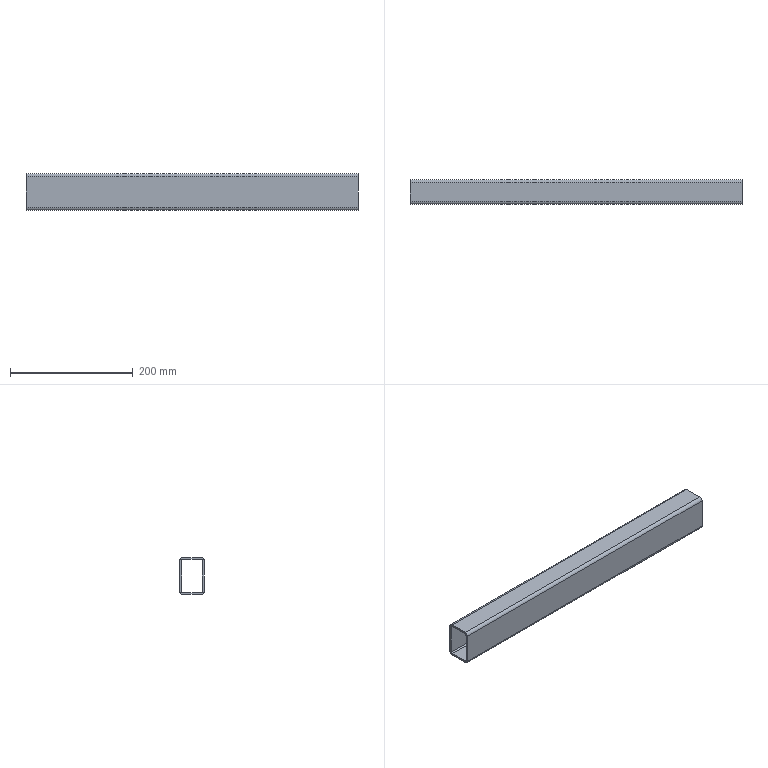Component | SolidWorks | THK-B1017FrontCrossBeam-2 | 1 solid | 22 faces | box 540 x 40 x 60 mm | volume 294774 mm3 | cylinder 12 | plane 10 | commonest cylinder face diameters 3.3 x4 10 x4 4 x4 | material Q235A
build123d program:
from build123d import *

# Parameters (mm, degrees)
EXTRUDE_THIN1_DEPTH   = 270
M4_TAPPED_HOLE1_D     = 3.3
M4_TAPPED_HOLE1_DEPTH = 3


with BuildPart() as part:
    # Sketch1 → Extrude-Thin1 (new, symmetric)
    with BuildSketch(Plane(origin=(0, 0, 0), x_dir=(0, 0, -1), z_dir=(1, 0, 0))):
        with BuildLine():
            Line((-30, 15), (-30, -15))
            ThreePointArc((-30, -15), (-28.536, -18.536), (-25, -20))
            Line((-25, -20), (25, -20))
            ThreePointArc((25, -20), (28.536, -18.536), (30, -15))
            Line((30, -15), (30, 15))
            ThreePointArc((30, 15), (28.536, 18.536), (25, 20))
            Line((25, 20), (-25, 20))
            ThreePointArc((-25, 20), (-28.536, 18.536), (-30, 15))
        make_face()
        with BuildLine():
            Line((-27, 15), (-27, -15))
            ThreePointArc((-27, -15), (-26.414, -16.414), (-25, -17))
            Line((-25, -17), (25, -17))
            ThreePointArc((25, -17), (26.414, -16.414), (27, -15))
            Line((27, -15), (27, 15))
            ThreePointArc((27, 15), (26.414, 16.414), (25, 17))
            Line((25, 17), (-25, 17))
            ThreePointArc((-25, 17), (-26.414, 16.414), (-27, 15))
        make_face(mode=Mode.SUBTRACT)
    extrude(amount=EXTRUDE_THIN1_DEPTH, both=True)

    # M4 Tapped Hole1
    with Locations(Plane(origin=(0, 20, 0), x_dir=(1, 0, 0), z_dir=(0, 1, 0))):
        with Locations((-150, 0), (-170, 0)):
            Hole(M4_TAPPED_HOLE1_D / 2, depth=M4_TAPPED_HOLE1_DEPTH)


solid = part.part

# Placed as in the assembly
solid = solid.moved(Location((0, -130, -860), (0, 0, 0)))
STEP:
#1=COLOUR_RGB('',0.7922,0.8196,0.9333);
#2=FILL_AREA_STYLE_COLOUR('',#1);
#3=FILL_AREA_STYLE('',(#2));
#4=SURFACE_STYLE_FILL_AREA(#3);
#5=SURFACE_SIDE_STYLE('',(#4));
#6=SURFACE_STYLE_USAGE(.BOTH.,#5);
#7=PRESENTATION_STYLE_ASSIGNMENT((#6));
#8=CARTESIAN_POINT('',(-5.906,-4.449,-33.793));
#9=VERTEX_POINT('',#8);
#10=CARTESIAN_POINT('',(-5.906,-4.449,-33.923));
#11=VERTEX_POINT('',#10);
#12=CARTESIAN_POINT('',(-5.906,-4.449,-33.858));
#13=DIRECTION('',(0.,-1.,0.));
#14=DIRECTION('',(0.,0.,-1.));
#15=AXIS2_PLACEMENT_3D('',#12,#13,#14);
#16=CIRCLE('',#15,0.06496);
#17=EDGE_CURVE('',#9,#11,#16,.T.);
#18=ORIENTED_EDGE('',*,*,#17,.T.);
#19=CARTESIAN_POINT('',(-5.906,-4.331,-33.923));
#20=VERTEX_POINT('',#19);
#21=CARTESIAN_POINT('',(-5.906,-4.331,-33.923));
#22=DIRECTION('',(0.,1.,0.));
#23=VECTOR('',#22,39.37);
#24=LINE('',#21,#23);
#25=EDGE_CURVE('',#11,#20,#24,.T.);
#26=ORIENTED_EDGE('',*,*,#25,.T.);
#27=CARTESIAN_POINT('',(-5.906,-4.331,-33.793));
#28=VERTEX_POINT('',#27);
#29=CARTESIAN_POINT('',(-5.906,-4.331,-33.858));
#30=DIRECTION('',(0.,1.,0.));
#31=DIRECTION('',(0.,0.,1.));
#32=AXIS2_PLACEMENT_3D('',#29,#30,#31);
#33=CIRCLE('',#32,0.06496);
#34=EDGE_CURVE('',#20,#28,#33,.T.);
#35=ORIENTED_EDGE('',*,*,#34,.T.);
#36=CARTESIAN_POINT('',(-5.906,-4.331,-33.793));
#37=DIRECTION('',(0.,1.,0.));
#38=VECTOR('',#37,39.37);
#39=LINE('',#36,#38);
#40=EDGE_CURVE('',#9,#28,#39,.T.);
#41=ORIENTED_EDGE('',*,*,#40,.F.);
#42=EDGE_LOOP('',(#18,#26,#35,#41));
#43=FACE_OUTER_BOUND('',#42,.T.);
#44=CARTESIAN_POINT('',(-5.906,-4.331,-33.858));
#45=DIRECTION('',(0.,1.,0.));
#46=DIRECTION('',(0.,0.,1.));
#47=AXIS2_PLACEMENT_3D('',#44,#45,#46);
#48=CYLINDRICAL_SURFACE('',#47,0.06496);
#49=ADVANCED_FACE('',(#43),#48,.F.);
#50=CARTESIAN_POINT('',(-6.693,-4.449,-33.793));
#51=VERTEX_POINT('',#50);
#52=CARTESIAN_POINT('',(-6.693,-4.449,-33.923));
#53=VERTEX_POINT('',#52);
#54=CARTESIAN_POINT('',(-6.693,-4.449,-33.858));
#55=DIRECTION('',(0.,-1.,0.));
#56=DIRECTION('',(0.,0.,-1.));
#57=AXIS2_PLACEMENT_3D('',#54,#55,#56);
#58=CIRCLE('',#57,0.06496);
#59=EDGE_CURVE('',#51,#53,#58,.T.);
#60=ORIENTED_EDGE('',*,*,#59,.T.);
#61=CARTESIAN_POINT('',(-6.693,-4.331,-33.923));
#62=VERTEX_POINT('',#61);
#63=CARTESIAN_POINT('',(-6.693,-4.331,-33.923));
#64=DIRECTION('',(0.,1.,0.));
#65=VECTOR('',#64,39.37);
#66=LINE('',#63,#65);
#67=EDGE_CURVE('',#53,#62,#66,.T.);
#68=ORIENTED_EDGE('',*,*,#67,.T.);
#69=CARTESIAN_POINT('',(-6.693,-4.331,-33.793));
#70=VERTEX_POINT('',#69);
#71=CARTESIAN_POINT('',(-6.693,-4.331,-33.858));
#72=DIRECTION('',(0.,1.,0.));
#73=DIRECTION('',(0.,0.,1.));
#74=AXIS2_PLACEMENT_3D('',#71,#72,#73);
#75=CIRCLE('',#74,0.06496);
#76=EDGE_CURVE('',#62,#70,#75,.T.);
#77=ORIENTED_EDGE('',*,*,#76,.T.);
#78=CARTESIAN_POINT('',(-6.693,-4.331,-33.793));
#79=DIRECTION('',(0.,1.,0.));
#80=VECTOR('',#79,39.37);
#81=LINE('',#78,#80);
#82=EDGE_CURVE('',#51,#70,#81,.T.);
#83=ORIENTED_EDGE('',*,*,#82,.F.);
#84=EDGE_LOOP('',(#60,#68,#77,#83));
#85=FACE_OUTER_BOUND('',#84,.T.);
#86=CARTESIAN_POINT('',(-6.693,-4.331,-33.858));
#87=DIRECTION('',(0.,1.,0.));
#88=DIRECTION('',(0.,0.,1.));
#89=AXIS2_PLACEMENT_3D('',#86,#87,#88);
#90=CYLINDRICAL_SURFACE('',#89,0.06496);
#91=ADVANCED_FACE('',(#85),#90,.F.);
#92=CARTESIAN_POINT('',(10.63,-5.709,-32.677));
#93=VERTEX_POINT('',#92);
#94=CARTESIAN_POINT('',(10.63,-5.906,-32.874));
#95=VERTEX_POINT('',#94);
#96=CARTESIAN_POINT('',(10.63,-5.709,-32.874));
#97=DIRECTION('',(1.,0.,0.));
#98=DIRECTION('',(0.,0.,-1.));
#99=AXIS2_PLACEMENT_3D('',#96,#97,#98);
#100=CIRCLE('',#99,0.1969);
#101=EDGE_CURVE('',#93,#95,#100,.T.);
#102=ORIENTED_EDGE('',*,*,#101,.T.);
#103=CARTESIAN_POINT('',(10.63,-5.906,-34.843));
#104=VERTEX_POINT('',#103);
#105=CARTESIAN_POINT('',(10.63,-5.906,-32.874));
#106=DIRECTION('',(0.,0.,-1.));
#107=VECTOR('',#106,39.37);
#108=LINE('',#105,#107);
#109=EDGE_CURVE('',#95,#104,#108,.T.);
#110=ORIENTED_EDGE('',*,*,#109,.T.);
#111=CARTESIAN_POINT('',(10.63,-5.709,-35.039));
#112=VERTEX_POINT('',#111);
#113=CARTESIAN_POINT('',(10.63,-5.709,-34.843));
#114=DIRECTION('',(1.,0.,0.));
#115=DIRECTION('',(0.,0.,1.));
#116=AXIS2_PLACEMENT_3D('',#113,#114,#115);
#117=CIRCLE('',#116,0.1969);
#118=EDGE_CURVE('',#104,#112,#117,.T.);
#119=ORIENTED_EDGE('',*,*,#118,.T.);
#120=CARTESIAN_POINT('',(10.63,-4.528,-35.039));
#121=VERTEX_POINT('',#120);
#122=CARTESIAN_POINT('',(10.63,-5.709,-35.039));
#123=DIRECTION('',(0.,1.,0.));
#124=VECTOR('',#123,39.37);
#125=LINE('',#122,#124);
#126=EDGE_CURVE('',#112,#121,#125,.T.);
#127=ORIENTED_EDGE('',*,*,#126,.T.);
#128=CARTESIAN_POINT('',(10.63,-4.331,-34.843));
#129=VERTEX_POINT('',#128);
#130=CARTESIAN_POINT('',(10.63,-4.528,-34.843));
#131=DIRECTION('',(1.,0.,0.));
#132=DIRECTION('',(0.,0.,-1.));
#133=AXIS2_PLACEMENT_3D('',#130,#131,#132);
#134=CIRCLE('',#133,0.1969);
#135=EDGE_CURVE('',#121,#129,#134,.T.);
#136=ORIENTED_EDGE('',*,*,#135,.T.);
#137=CARTESIAN_POINT('',(10.63,-4.331,-32.874));
#138=VERTEX_POINT('',#137);
#139=CARTESIAN_POINT('',(10.63,-4.331,-32.874));
#140=DIRECTION('',(0.,0.,1.));
#141=VECTOR('',#140,39.37);
#142=LINE('',#139,#141);
#143=EDGE_CURVE('',#129,#138,#142,.T.);
#144=ORIENTED_EDGE('',*,*,#143,.T.);
#145=CARTESIAN_POINT('',(10.63,-4.528,-32.677));
#146=VERTEX_POINT('',#145);
#147=CARTESIAN_POINT('',(10.63,-4.528,-32.874));
#148=DIRECTION('',(1.,0.,0.));
#149=DIRECTION('',(0.,0.,1.));
#150=AXIS2_PLACEMENT_3D('',#147,#148,#149);
#151=CIRCLE('',#150,0.1969);
#152=EDGE_CURVE('',#138,#146,#151,.T.);
#153=ORIENTED_EDGE('',*,*,#152,.T.);
#154=CARTESIAN_POINT('',(10.63,-5.709,-32.677));
#155=DIRECTION('',(0.,-1.,0.));
#156=VECTOR('',#155,39.37);
#157=LINE('',#154,#156);
#158=EDGE_CURVE('',#146,#93,#157,.T.);
#159=ORIENTED_EDGE('',*,*,#158,.T.);
#160=EDGE_LOOP('',(#102,#110,#119,#127,#136,#144,#153,#159));
#161=FACE_OUTER_BOUND('',#160,.T.);
#162=CARTESIAN_POINT('',(10.63,-5.787,-32.874));
#163=VERTEX_POINT('',#162);
#164=CARTESIAN_POINT('',(10.63,-5.787,-34.843));
#165=VERTEX_POINT('',#164);
#166=CARTESIAN_POINT('',(10.63,-5.787,-32.874));
#167=DIRECTION('',(0.,0.,-1.));
#168=VECTOR('',#167,39.37);
#169=LINE('',#166,#168);
#170=EDGE_CURVE('',#163,#165,#169,.T.);
#171=ORIENTED_EDGE('',*,*,#170,.F.);
#172=CARTESIAN_POINT('',(10.63,-5.709,-32.795));
#173=VERTEX_POINT('',#172);
#174=CARTESIAN_POINT('',(10.63,-5.709,-32.874));
#175=DIRECTION('',(1.,0.,0.));
#176=DIRECTION('',(0.,0.,-1.));
#177=AXIS2_PLACEMENT_3D('',#174,#175,#176);
#178=CIRCLE('',#177,0.07874);
#179=EDGE_CURVE('',#173,#163,#178,.T.);
#180=ORIENTED_EDGE('',*,*,#179,.F.);
#181=CARTESIAN_POINT('',(10.63,-4.528,-32.795));
#182=VERTEX_POINT('',#181);
#183=CARTESIAN_POINT('',(10.63,-5.709,-32.795));
#184=DIRECTION('',(0.,-1.,0.));
#185=VECTOR('',#184,39.37);
#186=LINE('',#183,#185);
#187=EDGE_CURVE('',#182,#173,#186,.T.);
#188=ORIENTED_EDGE('',*,*,#187,.F.);
#189=CARTESIAN_POINT('',(10.63,-4.449,-32.874));
#190=VERTEX_POINT('',#189);
#191=CARTESIAN_POINT('',(10.63,-4.528,-32.874));
#192=DIRECTION('',(1.,0.,0.));
#193=DIRECTION('',(0.,0.,-1.));
#194=AXIS2_PLACEMENT_3D('',#191,#192,#193);
#195=CIRCLE('',#194,0.07874);
#196=EDGE_CURVE('',#190,#182,#195,.T.);
#197=ORIENTED_EDGE('',*,*,#196,.F.);
#198=CARTESIAN_POINT('',(10.63,-4.449,-34.843));
#199=VERTEX_POINT('',#198);
#200=CARTESIAN_POINT('',(10.63,-4.449,-32.874));
#201=DIRECTION('',(0.,0.,1.));
#202=VECTOR('',#201,39.37);
#203=LINE('',#200,#202);
#204=EDGE_CURVE('',#199,#190,#203,.T.);
#205=ORIENTED_EDGE('',*,*,#204,.F.);
#206=CARTESIAN_POINT('',(10.63,-4.528,-34.921));
#207=VERTEX_POINT('',#206);
#208=CARTESIAN_POINT('',(10.63,-4.528,-34.843));
#209=DIRECTION('',(1.,0.,0.));
#210=DIRECTION('',(0.,0.,-1.));
#211=AXIS2_PLACEMENT_3D('',#208,#209,#210);
#212=CIRCLE('',#211,0.07874);
#213=EDGE_CURVE('',#207,#199,#212,.T.);
#214=ORIENTED_EDGE('',*,*,#213,.F.);
#215=CARTESIAN_POINT('',(10.63,-5.709,-34.921));
#216=VERTEX_POINT('',#215);
#217=CARTESIAN_POINT('',(10.63,-5.709,-34.921));
#218=DIRECTION('',(0.,1.,0.));
#219=VECTOR('',#218,39.37);
#220=LINE('',#217,#219);
#221=EDGE_CURVE('',#216,#207,#220,.T.);
#222=ORIENTED_EDGE('',*,*,#221,.F.);
#223=CARTESIAN_POINT('',(10.63,-5.709,-34.843));
#224=DIRECTION('',(1.,0.,0.));
#225=DIRECTION('',(0.,0.,-1.));
#226=AXIS2_PLACEMENT_3D('',#223,#224,#225);
#227=CIRCLE('',#226,0.07874);
#228=EDGE_CURVE('',#165,#216,#227,.T.);
#229=ORIENTED_EDGE('',*,*,#228,.F.);
#230=EDGE_LOOP('',(#171,#180,#188,#197,#205,#214,#222,#229));
#231=FACE_BOUND('',#230,.T.);
#232=CARTESIAN_POINT('',(10.63,-5.709,-32.874));
#233=DIRECTION('',(1.,0.,0.));
#234=DIRECTION('',(0.,0.,-1.));
#235=AXIS2_PLACEMENT_3D('',#232,#233,#234);
#236=PLANE('',#235);
#237=ADVANCED_FACE('',(#161,#231),#236,.T.);
#238=CARTESIAN_POINT('',(-10.63,-5.709,-32.677));
#239=VERTEX_POINT('',#238);
#240=CARTESIAN_POINT('',(-10.63,-5.906,-32.874));
#241=VERTEX_POINT('',#240);
#242=CARTESIAN_POINT('',(-10.63,-5.709,-32.874));
#243=DIRECTION('',(1.,0.,0.));
#244=DIRECTION('',(0.,0.,-1.));
#245=AXIS2_PLACEMENT_3D('',#242,#243,#244);
#246=CIRCLE('',#245,0.1969);
#247=EDGE_CURVE('',#239,#241,#246,.T.);
#248=ORIENTED_EDGE('',*,*,#247,.F.);
#249=CARTESIAN_POINT('',(-10.63,-4.528,-32.677));
#250=VERTEX_POINT('',#249);
#251=CARTESIAN_POINT('',(-10.63,-5.709,-32.677));
#252=DIRECTION('',(0.,-1.,0.));
#253=VECTOR('',#252,39.37);
#254=LINE('',#251,#253);
#255=EDGE_CURVE('',#250,#239,#254,.T.);
#256=ORIENTED_EDGE('',*,*,#255,.F.);
#257=CARTESIAN_POINT('',(-10.63,-4.331,-32.874));
#258=VERTEX_POINT('',#257);
#259=CARTESIAN_POINT('',(-10.63,-4.528,-32.874));
#260=DIRECTION('',(1.,0.,0.));
#261=DIRECTION('',(0.,0.,1.));
#262=AXIS2_PLACEMENT_3D('',#259,#260,#261);
#263=CIRCLE('',#262,0.1969);
#264=EDGE_CURVE('',#258,#250,#263,.T.);
#265=ORIENTED_EDGE('',*,*,#264,.F.);
#266=CARTESIAN_POINT('',(-10.63,-4.331,-34.843));
#267=VERTEX_POINT('',#266);
#268=CARTESIAN_POINT('',(-10.63,-4.331,-32.874));
#269=DIRECTION('',(0.,0.,1.));
#270=VECTOR('',#269,39.37);
#271=LINE('',#268,#270);
#272=EDGE_CURVE('',#267,#258,#271,.T.);
#273=ORIENTED_EDGE('',*,*,#272,.F.);
#274=CARTESIAN_POINT('',(-10.63,-4.528,-35.039));
#275=VERTEX_POINT('',#274);
#276=CARTESIAN_POINT('',(-10.63,-4.528,-34.843));
#277=DIRECTION('',(1.,0.,0.));
#278=DIRECTION('',(0.,0.,-1.));
#279=AXIS2_PLACEMENT_3D('',#276,#277,#278);
#280=CIRCLE('',#279,0.1969);
#281=EDGE_CURVE('',#275,#267,#280,.T.);
#282=ORIENTED_EDGE('',*,*,#281,.F.);
#283=CARTESIAN_POINT('',(-10.63,-5.709,-35.039));
#284=VERTEX_POINT('',#283);
#285=CARTESIAN_POINT('',(-10.63,-5.709,-35.039));
#286=DIRECTION('',(0.,1.,0.));
#287=VECTOR('',#286,39.37);
#288=LINE('',#285,#287);
#289=EDGE_CURVE('',#284,#275,#288,.T.);
#290=ORIENTED_EDGE('',*,*,#289,.F.);
#291=CARTESIAN_POINT('',(-10.63,-5.906,-34.843));
#292=VERTEX_POINT('',#291);
#293=CARTESIAN_POINT('',(-10.63,-5.709,-34.843));
#294=DIRECTION('',(1.,0.,0.));
#295=DIRECTION('',(0.,0.,1.));
#296=AXIS2_PLACEMENT_3D('',#293,#294,#295);
#297=CIRCLE('',#296,0.1969);
#298=EDGE_CURVE('',#292,#284,#297,.T.);
#299=ORIENTED_EDGE('',*,*,#298,.F.);
#300=CARTESIAN_POINT('',(-10.63,-5.906,-32.874));
#301=DIRECTION('',(0.,0.,-1.));
#302=VECTOR('',#301,39.37);
#303=LINE('',#300,#302);
#304=EDGE_CURVE('',#241,#292,#303,.T.);
#305=ORIENTED_EDGE('',*,*,#304,.F.);
#306=EDGE_LOOP('',(#248,#256,#265,#273,#282,#290,#299,#305));
#307=FACE_OUTER_BOUND('',#306,.T.);
#308=CARTESIAN_POINT('',(-10.63,-5.709,-32.795));
#309=VERTEX_POINT('',#308);
#310=CARTESIAN_POINT('',(-10.63,-5.787,-32.874));
#311=VERTEX_POINT('',#310);
#312=CARTESIAN_POINT('',(-10.63,-5.709,-32.874));
#313=DIRECTION('',(1.,0.,0.));
#314=DIRECTION('',(0.,0.,-1.));
#315=AXIS2_PLACEMENT_3D('',#312,#313,#314);
#316=CIRCLE('',#315,0.07874);
#317=EDGE_CURVE('',#309,#311,#316,.T.);
#318=ORIENTED_EDGE('',*,*,#317,.T.);
#319=CARTESIAN_POINT('',(-10.63,-5.787,-34.843));
#320=VERTEX_POINT('',#319);
#321=CARTESIAN_POINT('',(-10.63,-5.787,-32.874));
#322=DIRECTION('',(0.,0.,-1.));
#323=VECTOR('',#322,39.37);
#324=LINE('',#321,#323);
#325=EDGE_CURVE('',#311,#320,#324,.T.);
#326=ORIENTED_EDGE('',*,*,#325,.T.);
#327=CARTESIAN_POINT('',(-10.63,-5.709,-34.921));
#328=VERTEX_POINT('',#327);
#329=CARTESIAN_POINT('',(-10.63,-5.709,-34.843));
#330=DIRECTION('',(1.,0.,0.));
#331=DIRECTION('',(0.,0.,-1.));
#332=AXIS2_PLACEMENT_3D('',#329,#330,#331);
#333=CIRCLE('',#332,0.07874);
#334=EDGE_CURVE('',#320,#328,#333,.T.);
#335=ORIENTED_EDGE('',*,*,#334,.T.);
#336=CARTESIAN_POINT('',(-10.63,-4.528,-34.921));
#337=VERTEX_POINT('',#336);
#338=CARTESIAN_POINT('',(-10.63,-5.709,-34.921));
#339=DIRECTION('',(0.,1.,0.));
#340=VECTOR('',#339,39.37);
#341=LINE('',#338,#340);
#342=EDGE_CURVE('',#328,#337,#341,.T.);
#343=ORIENTED_EDGE('',*,*,#342,.T.);
#344=CARTESIAN_POINT('',(-10.63,-4.449,-34.843));
#345=VERTEX_POINT('',#344);
#346=CARTESIAN_POINT('',(-10.63,-4.528,-34.843));
#347=DIRECTION('',(1.,0.,0.));
#348=DIRECTION('',(0.,0.,-1.));
#349=AXIS2_PLACEMENT_3D('',#346,#347,#348);
#350=CIRCLE('',#349,0.07874);
#351=EDGE_CURVE('',#337,#345,#350,.T.);
#352=ORIENTED_EDGE('',*,*,#351,.T.);
#353=CARTESIAN_POINT('',(-10.63,-4.449,-32.874));
#354=VERTEX_POINT('',#353);
#355=CARTESIAN_POINT('',(-10.63,-4.449,-32.874));
#356=DIRECTION('',(0.,0.,1.));
#357=VECTOR('',#356,39.37);
#358=LINE('',#355,#357);
#359=EDGE_CURVE('',#345,#354,#358,.T.);
#360=ORIENTED_EDGE('',*,*,#359,.T.);
#361=CARTESIAN_POINT('',(-10.63,-4.528,-32.795));
#362=VERTEX_POINT('',#361);
#363=CARTESIAN_POINT('',(-10.63,-4.528,-32.874));
#364=DIRECTION('',(1.,0.,0.));
#365=DIRECTION('',(0.,0.,-1.));
#366=AXIS2_PLACEMENT_3D('',#363,#364,#365);
#367=CIRCLE('',#366,0.07874);
#368=EDGE_CURVE('',#354,#362,#367,.T.);
#369=ORIENTED_EDGE('',*,*,#368,.T.);
#370=CARTESIAN_POINT('',(-10.63,-5.709,-32.795));
#371=DIRECTION('',(0.,-1.,0.));
#372=VECTOR('',#371,39.37);
#373=LINE('',#370,#372);
#374=EDGE_CURVE('',#362,#309,#373,.T.);
#375=ORIENTED_EDGE('',*,*,#374,.T.);
#376=EDGE_LOOP('',(#318,#326,#335,#343,#352,#360,#369,#375));
#377=FACE_BOUND('',#376,.T.);
#378=CARTESIAN_POINT('',(-10.63,-5.709,-32.874));
#379=DIRECTION('',(1.,0.,0.));
#380=DIRECTION('',(0.,0.,-1.));
#381=AXIS2_PLACEMENT_3D('',#378,#379,#380);
#382=PLANE('',#381);
#383=ADVANCED_FACE('',(#307,#377),#382,.F.);
#384=ORIENTED_EDGE('',*,*,#247,.T.);
#385=CARTESIAN_POINT('',(10.63,-5.906,-32.874));
#386=DIRECTION('',(-1.,0.,0.));
#387=VECTOR('',#386,39.37);
#388=LINE('',#385,#387);
#389=EDGE_CURVE('',#95,#241,#388,.T.);
#390=ORIENTED_EDGE('',*,*,#389,.F.);
#391=ORIENTED_EDGE('',*,*,#101,.F.);
#392=CARTESIAN_POINT('',(10.63,-5.709,-32.677));
#393=DIRECTION('',(-1.,0.,0.));
#394=VECTOR('',#393,39.37);
#395=LINE('',#392,#394);
#396=EDGE_CURVE('',#93,#239,#395,.T.);
#397=ORIENTED_EDGE('',*,*,#396,.T.);
#398=EDGE_LOOP('',(#384,#390,#391,#397));
#399=FACE_OUTER_BOUND('',#398,.T.);
#400=CARTESIAN_POINT('',(10.63,-5.709,-32.874));
#401=DIRECTION('',(-1.,0.,0.));
#402=DIRECTION('',(0.,0.,1.));
#403=AXIS2_PLACEMENT_3D('',#400,#401,#402);
#404=CYLINDRICAL_SURFACE('',#403,0.1969);
#405=ADVANCED_FACE('',(#399),#404,.T.);
#406=ORIENTED_EDGE('',*,*,#304,.T.);
#407=CARTESIAN_POINT('',(10.63,-5.906,-34.843));
#408=DIRECTION('',(-1.,0.,0.));
#409=VECTOR('',#408,39.37);
#410=LINE('',#407,#409);
#411=EDGE_CURVE('',#104,#292,#410,.T.);
#412=ORIENTED_EDGE('',*,*,#411,.F.);
#413=ORIENTED_EDGE('',*,*,#109,.F.);
#414=ORIENTED_EDGE('',*,*,#389,.T.);
#415=EDGE_LOOP('',(#406,#412,#413,#414));
#416=FACE_OUTER_BOUND('',#415,.T.);
#417=CARTESIAN_POINT('',(10.63,-5.906,-32.874));
#418=DIRECTION('',(0.,1.,0.));
#419=DIRECTION('',(0.,0.,1.));
#420=AXIS2_PLACEMENT_3D('',#417,#418,#419);
#421=PLANE('',#420);
#422=ADVANCED_FACE('',(#416),#421,.F.);
#423=ORIENTED_EDGE('',*,*,#298,.T.);
#424=CARTESIAN_POINT('',(10.63,-5.709,-35.039));
#425=DIRECTION('',(-1.,0.,0.));
#426=VECTOR('',#425,39.37);
#427=LINE('',#424,#426);
#428=EDGE_CURVE('',#112,#284,#427,.T.);
#429=ORIENTED_EDGE('',*,*,#428,.F.);
#430=ORIENTED_EDGE('',*,*,#118,.F.);
#431=ORIENTED_EDGE('',*,*,#411,.T.);
#432=EDGE_LOOP('',(#423,#429,#430,#431));
#433=FACE_OUTER_BOUND('',#432,.T.);
#434=CARTESIAN_POINT('',(10.63,-5.709,-34.843));
#435=DIRECTION('',(-1.,0.,0.));
#436=DIRECTION('',(0.,0.,1.));
#437=AXIS2_PLACEMENT_3D('',#434,#435,#436);
#438=CYLINDRICAL_SURFACE('',#437,0.1969);
#439=ADVANCED_FACE('',(#433),#438,.T.);
#440=ORIENTED_EDGE('',*,*,#289,.T.);
#441=CARTESIAN_POINT('',(10.63,-4.528,-35.039));
#442=DIRECTION('',(-1.,0.,0.));
#443=VECTOR('',#442,39.37);
#444=LINE('',#441,#443);
#445=EDGE_CURVE('',#121,#275,#444,.T.);
#446=ORIENTED_EDGE('',*,*,#445,.F.);
#447=ORIENTED_EDGE('',*,*,#126,.F.);
#448=ORIENTED_EDGE('',*,*,#428,.T.);
#449=EDGE_LOOP('',(#440,#446,#447,#448));
#450=FACE_OUTER_BOUND('',#449,.T.);
#451=CARTESIAN_POINT('',(10.63,-5.709,-35.039));
#452=DIRECTION('',(0.,0.,1.));
#453=DIRECTION('',(1.,0.,0.));
#454=AXIS2_PLACEMENT_3D('',#451,#452,#453);
#455=PLANE('',#454);
#456=ADVANCED_FACE('',(#450),#455,.F.);
#457=ORIENTED_EDGE('',*,*,#281,.T.);
#458=CARTESIAN_POINT('',(10.63,-4.331,-34.843));
#459=DIRECTION('',(-1.,0.,0.));
#460=VECTOR('',#459,39.37);
#461=LINE('',#458,#460);
#462=EDGE_CURVE('',#129,#267,#461,.T.);
#463=ORIENTED_EDGE('',*,*,#462,.F.);
#464=ORIENTED_EDGE('',*,*,#135,.F.);
#465=ORIENTED_EDGE('',*,*,#445,.T.);
#466=EDGE_LOOP('',(#457,#463,#464,#465));
#467=FACE_OUTER_BOUND('',#466,.T.);
#468=CARTESIAN_POINT('',(10.63,-4.528,-34.843));
#469=DIRECTION('',(-1.,0.,0.));
#470=DIRECTION('',(0.,0.,1.));
#471=AXIS2_PLACEMENT_3D('',#468,#469,#470);
#472=CYLINDRICAL_SURFACE('',#471,0.1969);
#473=ADVANCED_FACE('',(#467),#472,.T.);
#474=CARTESIAN_POINT('',(-5.906,-4.331,-33.858));
#475=DIRECTION('',(0.,1.,0.));
#476=DIRECTION('',(0.,0.,1.));
#477=AXIS2_PLACEMENT_3D('',#474,#475,#476);
#478=CIRCLE('',#477,0.06496);
#479=EDGE_CURVE('',#28,#20,#478,.T.);
#480=ORIENTED_EDGE('',*,*,#479,.F.);
#481=ORIENTED_EDGE('',*,*,#34,.F.);
#482=EDGE_LOOP('',(#480,#481));
#483=FACE_BOUND('',#482,.T.);
#484=CARTESIAN_POINT('',(-6.693,-4.331,-33.858));
#485=DIRECTION('',(0.,1.,0.));
#486=DIRECTION('',(0.,0.,1.));
#487=AXIS2_PLACEMENT_3D('',#484,#485,#486);
#488=CIRCLE('',#487,0.06496);
#489=EDGE_CURVE('',#70,#62,#488,.T.);
#490=ORIENTED_EDGE('',*,*,#489,.F.);
#491=ORIENTED_EDGE('',*,*,#76,.F.);
#492=EDGE_LOOP('',(#490,#491));
#493=FACE_BOUND('',#492,.T.);
#494=ORIENTED_EDGE('',*,*,#272,.T.);
#495=CARTESIAN_POINT('',(10.63,-4.331,-32.874));
#496=DIRECTION('',(-1.,0.,0.));
#497=VECTOR('',#496,39.37);
#498=LINE('',#495,#497);
#499=EDGE_CURVE('',#138,#258,#498,.T.);
#500=ORIENTED_EDGE('',*,*,#499,.F.);
#501=ORIENTED_EDGE('',*,*,#143,.F.);
#502=ORIENTED_EDGE('',*,*,#462,.T.);
#503=EDGE_LOOP('',(#494,#500,#501,#502));
#504=FACE_OUTER_BOUND('',#503,.T.);
#505=CARTESIAN_POINT('',(10.63,-4.331,-32.874));
#506=DIRECTION('',(0.,-1.,0.));
#507=DIRECTION('',(0.,0.,-1.));
#508=AXIS2_PLACEMENT_3D('',#505,#506,#507);
#509=PLANE('',#508);
#510=ADVANCED_FACE('',(#483,#493,#504),#509,.F.);
#511=ORIENTED_EDGE('',*,*,#264,.T.);
#512=CARTESIAN_POINT('',(10.63,-4.528,-32.677));
#513=DIRECTION('',(-1.,0.,0.));
#514=VECTOR('',#513,39.37);
#515=LINE('',#512,#514);
#516=EDGE_CURVE('',#146,#250,#515,.T.);
#517=ORIENTED_EDGE('',*,*,#516,.F.);
#518=ORIENTED_EDGE('',*,*,#152,.F.);
#519=ORIENTED_EDGE('',*,*,#499,.T.);
#520=EDGE_LOOP('',(#511,#517,#518,#519));
#521=FACE_OUTER_BOUND('',#520,.T.);
#522=CARTESIAN_POINT('',(10.63,-4.528,-32.874));
#523=DIRECTION('',(-1.,0.,0.));
#524=DIRECTION('',(0.,0.,1.));
#525=AXIS2_PLACEMENT_3D('',#522,#523,#524);
#526=CYLINDRICAL_SURFACE('',#525,0.1969);
#527=ADVANCED_FACE('',(#521),#526,.T.);
#528=ORIENTED_EDGE('',*,*,#255,.T.);
#529=ORIENTED_EDGE('',*,*,#396,.F.);
#530=ORIENTED_EDGE('',*,*,#158,.F.);
#531=ORIENTED_EDGE('',*,*,#516,.T.);
#532=EDGE_LOOP('',(#528,#529,#530,#531));
#533=FACE_OUTER_BOUND('',#532,.T.);
#534=CARTESIAN_POINT('',(10.63,-5.709,-32.677));
#535=DIRECTION('',(0.,0.,-1.));
#536=DIRECTION('',(-1.,0.,0.));
#537=AXIS2_PLACEMENT_3D('',#534,#535,#536);
#538=PLANE('',#537);
#539=ADVANCED_FACE('',(#533),#538,.F.);
#540=ORIENTED_EDGE('',*,*,#317,.F.);
#541=CARTESIAN_POINT('',(10.63,-5.709,-32.795));
#542=DIRECTION('',(-1.,0.,0.));
#543=VECTOR('',#542,39.37);
#544=LINE('',#541,#543);
#545=EDGE_CURVE('',#173,#309,#544,.T.);
#546=ORIENTED_EDGE('',*,*,#545,.F.);
#547=ORIENTED_EDGE('',*,*,#179,.T.);
#548=CARTESIAN_POINT('',(10.63,-5.787,-32.874));
#549=DIRECTION('',(-1.,0.,0.));
#550=VECTOR('',#549,39.37);
#551=LINE('',#548,#550);
#552=EDGE_CURVE('',#163,#311,#551,.T.);
#553=ORIENTED_EDGE('',*,*,#552,.T.);
#554=EDGE_LOOP('',(#540,#546,#547,#553));
#555=FACE_OUTER_BOUND('',#554,.T.);
#556=CARTESIAN_POINT('',(10.63,-5.709,-32.874));
#557=DIRECTION('',(-1.,0.,0.));
#558=DIRECTION('',(0.,0.,1.));
#559=AXIS2_PLACEMENT_3D('',#556,#557,#558);
#560=CYLINDRICAL_SURFACE('',#559,0.07874);
#561=ADVANCED_FACE('',(#555),#560,.F.);
#562=ORIENTED_EDGE('',*,*,#325,.F.);
#563=ORIENTED_EDGE('',*,*,#552,.F.);
#564=ORIENTED_EDGE('',*,*,#170,.T.);
#565=CARTESIAN_POINT('',(10.63,-5.787,-34.843));
#566=DIRECTION('',(-1.,0.,0.));
#567=VECTOR('',#566,39.37);
#568=LINE('',#565,#567);
#569=EDGE_CURVE('',#165,#320,#568,.T.);
#570=ORIENTED_EDGE('',*,*,#569,.T.);
#571=EDGE_LOOP('',(#562,#563,#564,#570));
#572=FACE_OUTER_BOUND('',#571,.T.);
#573=CARTESIAN_POINT('',(10.63,-5.787,-32.874));
#574=DIRECTION('',(0.,1.,0.));
#575=DIRECTION('',(0.,0.,1.));
#576=AXIS2_PLACEMENT_3D('',#573,#574,#575);
#577=PLANE('',#576);
#578=ADVANCED_FACE('',(#572),#577,.T.);
#579=ORIENTED_EDGE('',*,*,#334,.F.);
#580=ORIENTED_EDGE('',*,*,#569,.F.);
#581=ORIENTED_EDGE('',*,*,#228,.T.);
#582=CARTESIAN_POINT('',(10.63,-5.709,-34.921));
#583=DIRECTION('',(-1.,0.,0.));
#584=VECTOR('',#583,39.37);
#585=LINE('',#582,#584);
#586=EDGE_CURVE('',#216,#328,#585,.T.);
#587=ORIENTED_EDGE('',*,*,#586,.T.);
#588=EDGE_LOOP('',(#579,#580,#581,#587));
#589=FACE_OUTER_BOUND('',#588,.T.);
#590=CARTESIAN_POINT('',(10.63,-5.709,-34.843));
#591=DIRECTION('',(-1.,0.,0.));
#592=DIRECTION('',(0.,0.,1.));
#593=AXIS2_PLACEMENT_3D('',#590,#591,#592);
#594=CYLINDRICAL_SURFACE('',#593,0.07874);
#595=ADVANCED_FACE('',(#589),#594,.F.);
#596=ORIENTED_EDGE('',*,*,#342,.F.);
#597=ORIENTED_EDGE('',*,*,#586,.F.);
#598=ORIENTED_EDGE('',*,*,#221,.T.);
#599=CARTESIAN_POINT('',(10.63,-4.528,-34.921));
#600=DIRECTION('',(-1.,0.,0.));
#601=VECTOR('',#600,39.37);
#602=LINE('',#599,#601);
#603=EDGE_CURVE('',#207,#337,#602,.T.);
#604=ORIENTED_EDGE('',*,*,#603,.T.);
#605=EDGE_LOOP('',(#596,#597,#598,#604));
#606=FACE_OUTER_BOUND('',#605,.T.);
#607=CARTESIAN_POINT('',(10.63,-5.709,-34.921));
#608=DIRECTION('',(0.,0.,1.));
#609=DIRECTION('',(1.,0.,0.));
#610=AXIS2_PLACEMENT_3D('',#607,#608,#609);
#611=PLANE('',#610);
#612=ADVANCED_FACE('',(#606),#611,.T.);
#613=ORIENTED_EDGE('',*,*,#351,.F.);
#614=ORIENTED_EDGE('',*,*,#603,.F.);
#615=ORIENTED_EDGE('',*,*,#213,.T.);
#616=CARTESIAN_POINT('',(10.63,-4.449,-34.843));
#617=DIRECTION('',(-1.,0.,0.));
#618=VECTOR('',#617,39.37);
#619=LINE('',#616,#618);
#620=EDGE_CURVE('',#199,#345,#619,.T.);
#621=ORIENTED_EDGE('',*,*,#620,.T.);
#622=EDGE_LOOP('',(#613,#614,#615,#621));
#623=FACE_OUTER_BOUND('',#622,.T.);
#624=CARTESIAN_POINT('',(10.63,-4.528,-34.843));
#625=DIRECTION('',(-1.,0.,0.));
#626=DIRECTION('',(0.,0.,1.));
#627=AXIS2_PLACEMENT_3D('',#624,#625,#626);
#628=CYLINDRICAL_SURFACE('',#627,0.07874);
#629=ADVANCED_FACE('',(#623),#628,.F.);
#630=ORIENTED_EDGE('',*,*,#17,.F.);
#631=CARTESIAN_POINT('',(-5.906,-4.449,-33.858));
#632=DIRECTION('',(0.,-1.,0.));
#633=DIRECTION('',(0.,0.,-1.));
#634=AXIS2_PLACEMENT_3D('',#631,#632,#633);
#635=CIRCLE('',#634,0.06496);
#636=EDGE_CURVE('',#11,#9,#635,.T.);
#637=ORIENTED_EDGE('',*,*,#636,.F.);
#638=EDGE_LOOP('',(#630,#637));
#639=FACE_BOUND('',#638,.T.);
#640=ORIENTED_EDGE('',*,*,#59,.F.);
#641=CARTESIAN_POINT('',(-6.693,-4.449,-33.858));
#642=DIRECTION('',(0.,-1.,0.));
#643=DIRECTION('',(0.,0.,-1.));
#644=AXIS2_PLACEMENT_3D('',#641,#642,#643);
#645=CIRCLE('',#644,0.06496);
#646=EDGE_CURVE('',#53,#51,#645,.T.);
#647=ORIENTED_EDGE('',*,*,#646,.F.);
#648=EDGE_LOOP('',(#640,#647));
#649=FACE_BOUND('',#648,.T.);
#650=ORIENTED_EDGE('',*,*,#359,.F.);
#651=ORIENTED_EDGE('',*,*,#620,.F.);
#652=ORIENTED_EDGE('',*,*,#204,.T.);
#653=CARTESIAN_POINT('',(10.63,-4.449,-32.874));
#654=DIRECTION('',(-1.,0.,0.));
#655=VECTOR('',#654,39.37);
#656=LINE('',#653,#655);
#657=EDGE_CURVE('',#190,#354,#656,.T.);
#658=ORIENTED_EDGE('',*,*,#657,.T.);
#659=EDGE_LOOP('',(#650,#651,#652,#658));
#660=FACE_OUTER_BOUND('',#659,.T.);
#661=CARTESIAN_POINT('',(10.63,-4.449,-32.874));
#662=DIRECTION('',(0.,-1.,0.));
#663=DIRECTION('',(0.,0.,-1.));
#664=AXIS2_PLACEMENT_3D('',#661,#662,#663);
#665=PLANE('',#664);
#666=ADVANCED_FACE('',(#639,#649,#660),#665,.T.);
#667=ORIENTED_EDGE('',*,*,#368,.F.);
#668=ORIENTED_EDGE('',*,*,#657,.F.);
#669=ORIENTED_EDGE('',*,*,#196,.T.);
#670=CARTESIAN_POINT('',(10.63,-4.528,-32.795));
#671=DIRECTION('',(-1.,0.,0.));
#672=VECTOR('',#671,39.37);
#673=LINE('',#670,#672);
#674=EDGE_CURVE('',#182,#362,#673,.T.);
#675=ORIENTED_EDGE('',*,*,#674,.T.);
#676=EDGE_LOOP('',(#667,#668,#669,#675));
#677=FACE_OUTER_BOUND('',#676,.T.);
#678=CARTESIAN_POINT('',(10.63,-4.528,-32.874));
#679=DIRECTION('',(-1.,0.,0.));
#680=DIRECTION('',(0.,0.,1.));
#681=AXIS2_PLACEMENT_3D('',#678,#679,#680);
#682=CYLINDRICAL_SURFACE('',#681,0.07874);
#683=ADVANCED_FACE('',(#677),#682,.F.);
#684=ORIENTED_EDGE('',*,*,#374,.F.);
#685=ORIENTED_EDGE('',*,*,#674,.F.);
#686=ORIENTED_EDGE('',*,*,#187,.T.);
#687=ORIENTED_EDGE('',*,*,#545,.T.);
#688=EDGE_LOOP('',(#684,#685,#686,#687));
#689=FACE_OUTER_BOUND('',#688,.T.);
#690=CARTESIAN_POINT('',(10.63,-5.709,-32.795));
#691=DIRECTION('',(0.,0.,-1.));
#692=DIRECTION('',(-1.,0.,0.));
#693=AXIS2_PLACEMENT_3D('',#690,#691,#692);
#694=PLANE('',#693);
#695=ADVANCED_FACE('',(#689),#694,.T.);
#696=ORIENTED_EDGE('',*,*,#67,.F.);
#697=ORIENTED_EDGE('',*,*,#646,.T.);
#698=ORIENTED_EDGE('',*,*,#82,.T.);
#699=ORIENTED_EDGE('',*,*,#489,.T.);
#700=EDGE_LOOP('',(#696,#697,#698,#699));
#701=FACE_OUTER_BOUND('',#700,.T.);
#702=CARTESIAN_POINT('',(-6.693,-4.331,-33.858));
#703=DIRECTION('',(0.,1.,0.));
#704=DIRECTION('',(0.,0.,1.));
#705=AXIS2_PLACEMENT_3D('',#702,#703,#704);
#706=CYLINDRICAL_SURFACE('',#705,0.06496);
#707=ADVANCED_FACE('',(#701),#706,.F.);
#708=ORIENTED_EDGE('',*,*,#25,.F.);
#709=ORIENTED_EDGE('',*,*,#636,.T.);
#710=ORIENTED_EDGE('',*,*,#40,.T.);
#711=ORIENTED_EDGE('',*,*,#479,.T.);
#712=EDGE_LOOP('',(#708,#709,#710,#711));
#713=FACE_OUTER_BOUND('',#712,.T.);
#714=CARTESIAN_POINT('',(-5.906,-4.331,-33.858));
#715=DIRECTION('',(0.,1.,0.));
#716=DIRECTION('',(0.,0.,1.));
#717=AXIS2_PLACEMENT_3D('',#714,#715,#716);
#718=CYLINDRICAL_SURFACE('',#717,0.06496);
#719=ADVANCED_FACE('',(#713),#718,.F.);
#720=CLOSED_SHELL('',(#49,#91,#237,#383,#405,#422,#439,#456,#473,#510,#527,#539,#561,#578,#595,#612,#629,#666,#683,#695,#707,#719));
#721=MANIFOLD_SOLID_BREP('',#720);
#722=STYLED_ITEM('',(#7),#721);
#723=(LENGTH_UNIT()NAMED_UNIT(*)SI_UNIT($,.METRE.));
#724=LENGTH_MEASURE_WITH_UNIT(LENGTH_MEASURE(0.0254),#723);
#725=DIMENSIONAL_EXPONENTS(1.,0.,0.,0.,0.,0.,0.);
#726=(CONVERSION_BASED_UNIT('',#724)LENGTH_UNIT()NAMED_UNIT(#725));
#727=UNCERTAINTY_MEASURE_WITH_UNIT(LENGTH_MEASURE(0.00001),#726,'','');
#728=(NAMED_UNIT(*)PLANE_ANGLE_UNIT()SI_UNIT($,.RADIAN.));
#729=(NAMED_UNIT(*)SI_UNIT($,.STERADIAN.)SOLID_ANGLE_UNIT());
#730=(GEOMETRIC_REPRESENTATION_CONTEXT(3)GLOBAL_UNCERTAINTY_ASSIGNED_CONTEXT((#727))GLOBAL_UNIT_ASSIGNED_CONTEXT((#726,#728,#729))REPRESENTATION_CONTEXT('',''));
#731=MECHANICAL_DESIGN_GEOMETRIC_PRESENTATION_REPRESENTATION('',(#722),#730);
#732=CARTESIAN_POINT('',(0.,0.,0.));
#733=DIRECTION('',(0.,0.,1.));
#734=DIRECTION('',(1.,0.,0.));
#735=AXIS2_PLACEMENT_3D('',#732,#733,#734);
#736=(LENGTH_UNIT()NAMED_UNIT(*)SI_UNIT($,.METRE.));
#737=LENGTH_MEASURE_WITH_UNIT(LENGTH_MEASURE(0.0254),#736);
#738=DIMENSIONAL_EXPONENTS(1.,0.,0.,0.,0.,0.,0.);
#739=(CONVERSION_BASED_UNIT('',#737)LENGTH_UNIT()NAMED_UNIT(#738));
#740=UNCERTAINTY_MEASURE_WITH_UNIT(LENGTH_MEASURE(0.00001),#739,'','');
#741=(NAMED_UNIT(*)PLANE_ANGLE_UNIT()SI_UNIT($,.RADIAN.));
#742=(NAMED_UNIT(*)SI_UNIT($,.STERADIAN.)SOLID_ANGLE_UNIT());
#743=(GEOMETRIC_REPRESENTATION_CONTEXT(3)GLOBAL_UNCERTAINTY_ASSIGNED_CONTEXT((#740))GLOBAL_UNIT_ASSIGNED_CONTEXT((#739,#741,#742))REPRESENTATION_CONTEXT('',''));
#744=ADVANCED_BREP_SHAPE_REPRESENTATION('',(#721,#735),#743);
#745=PRESENTATION_LAYER_ASSIGNMENT('','',(#722));